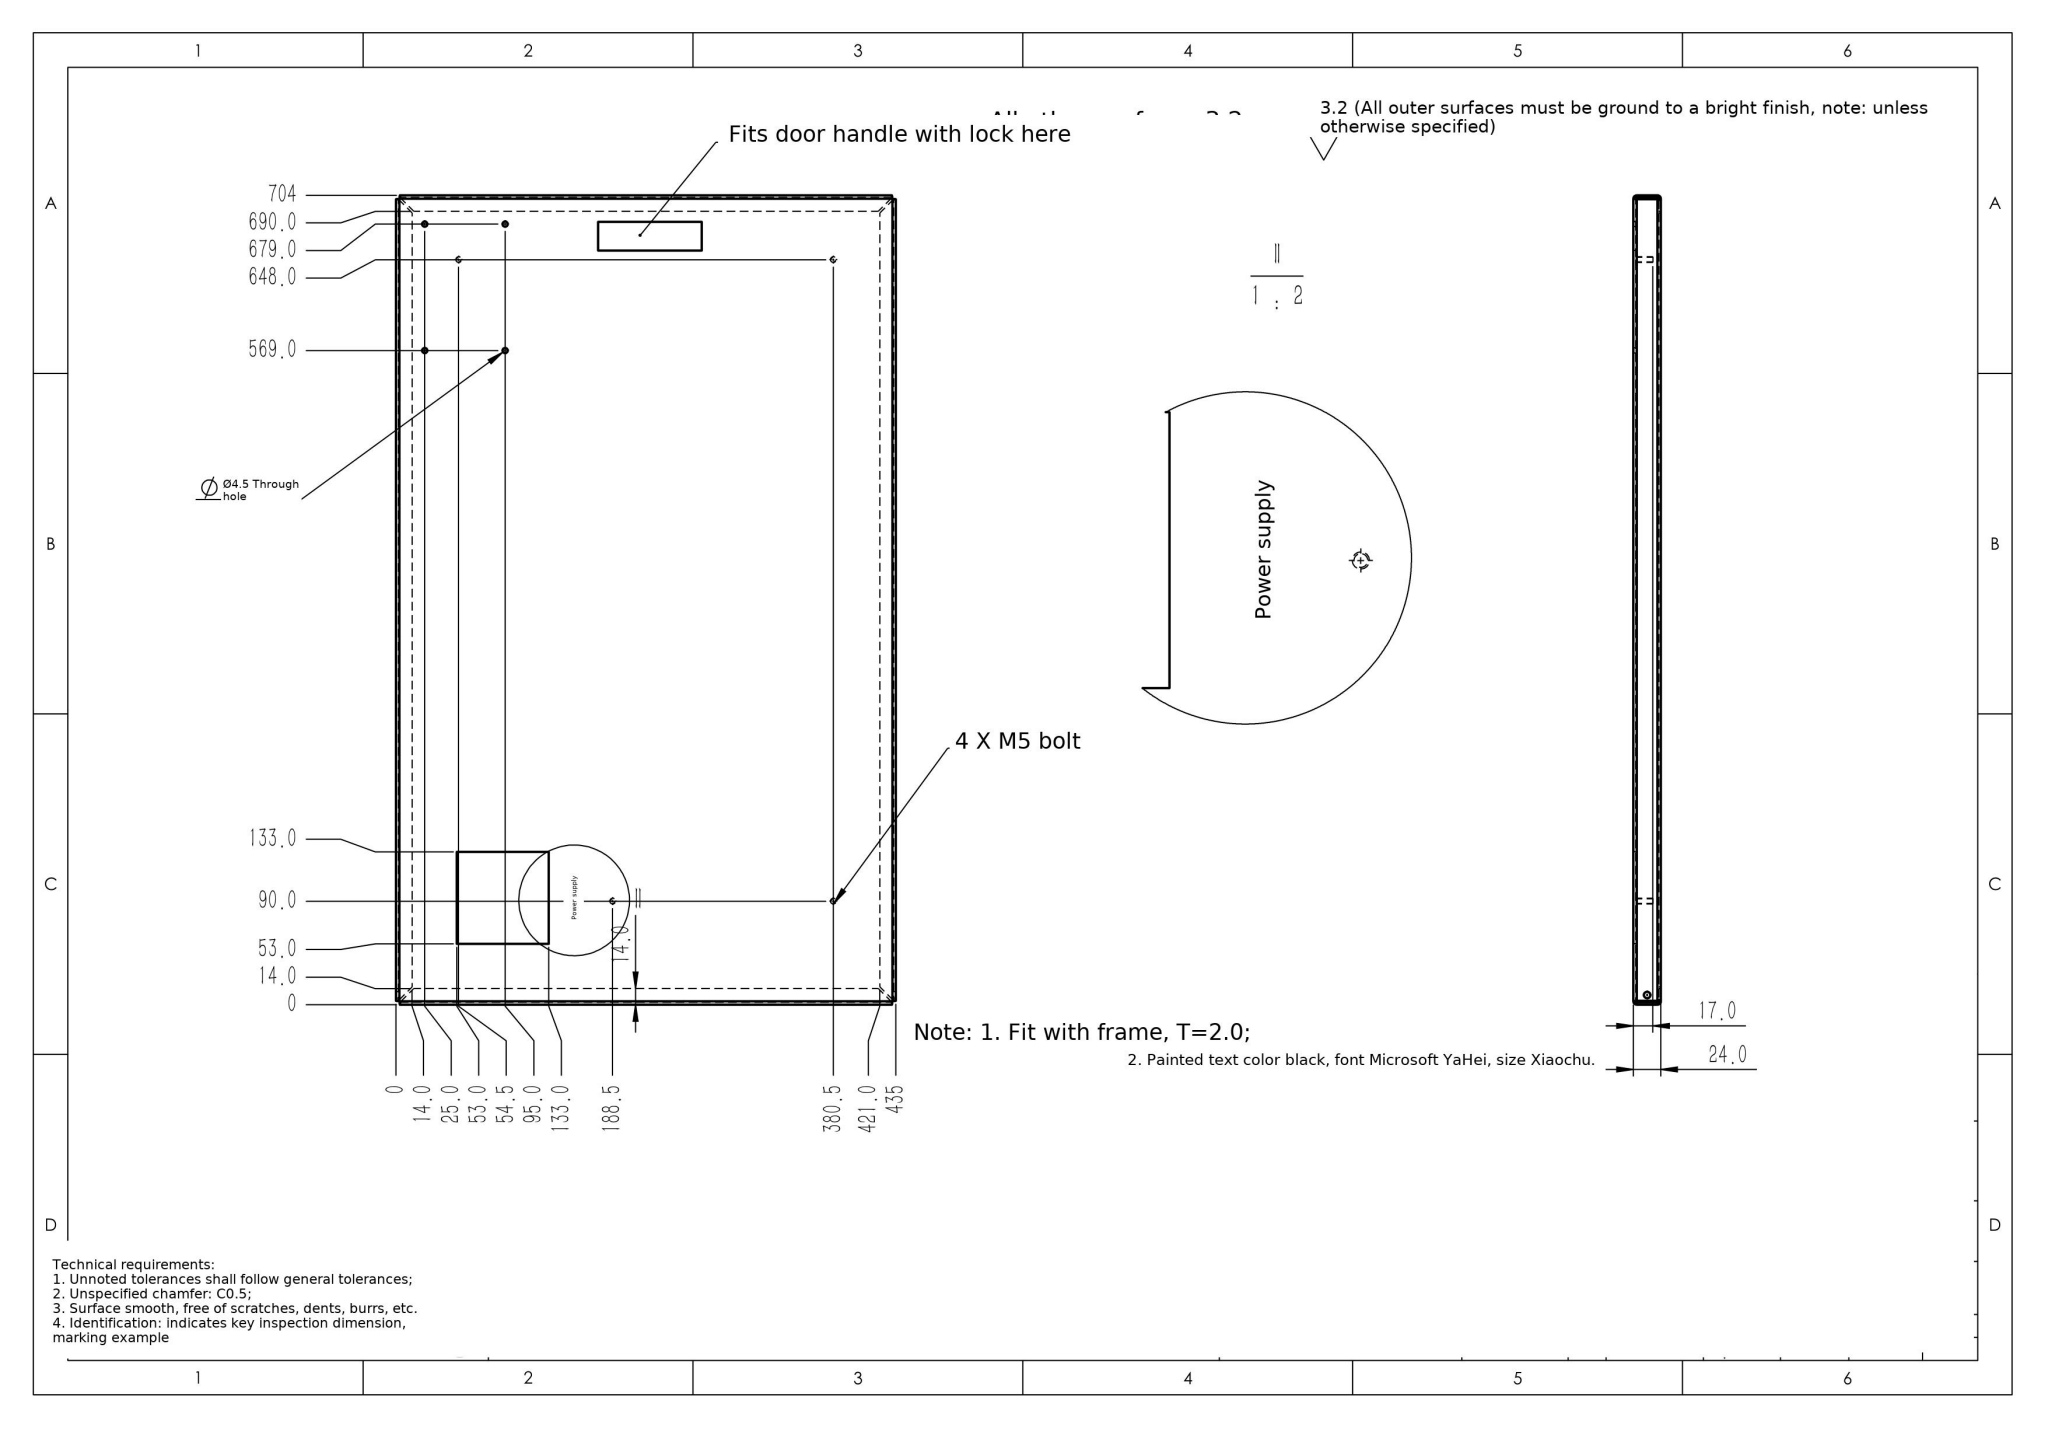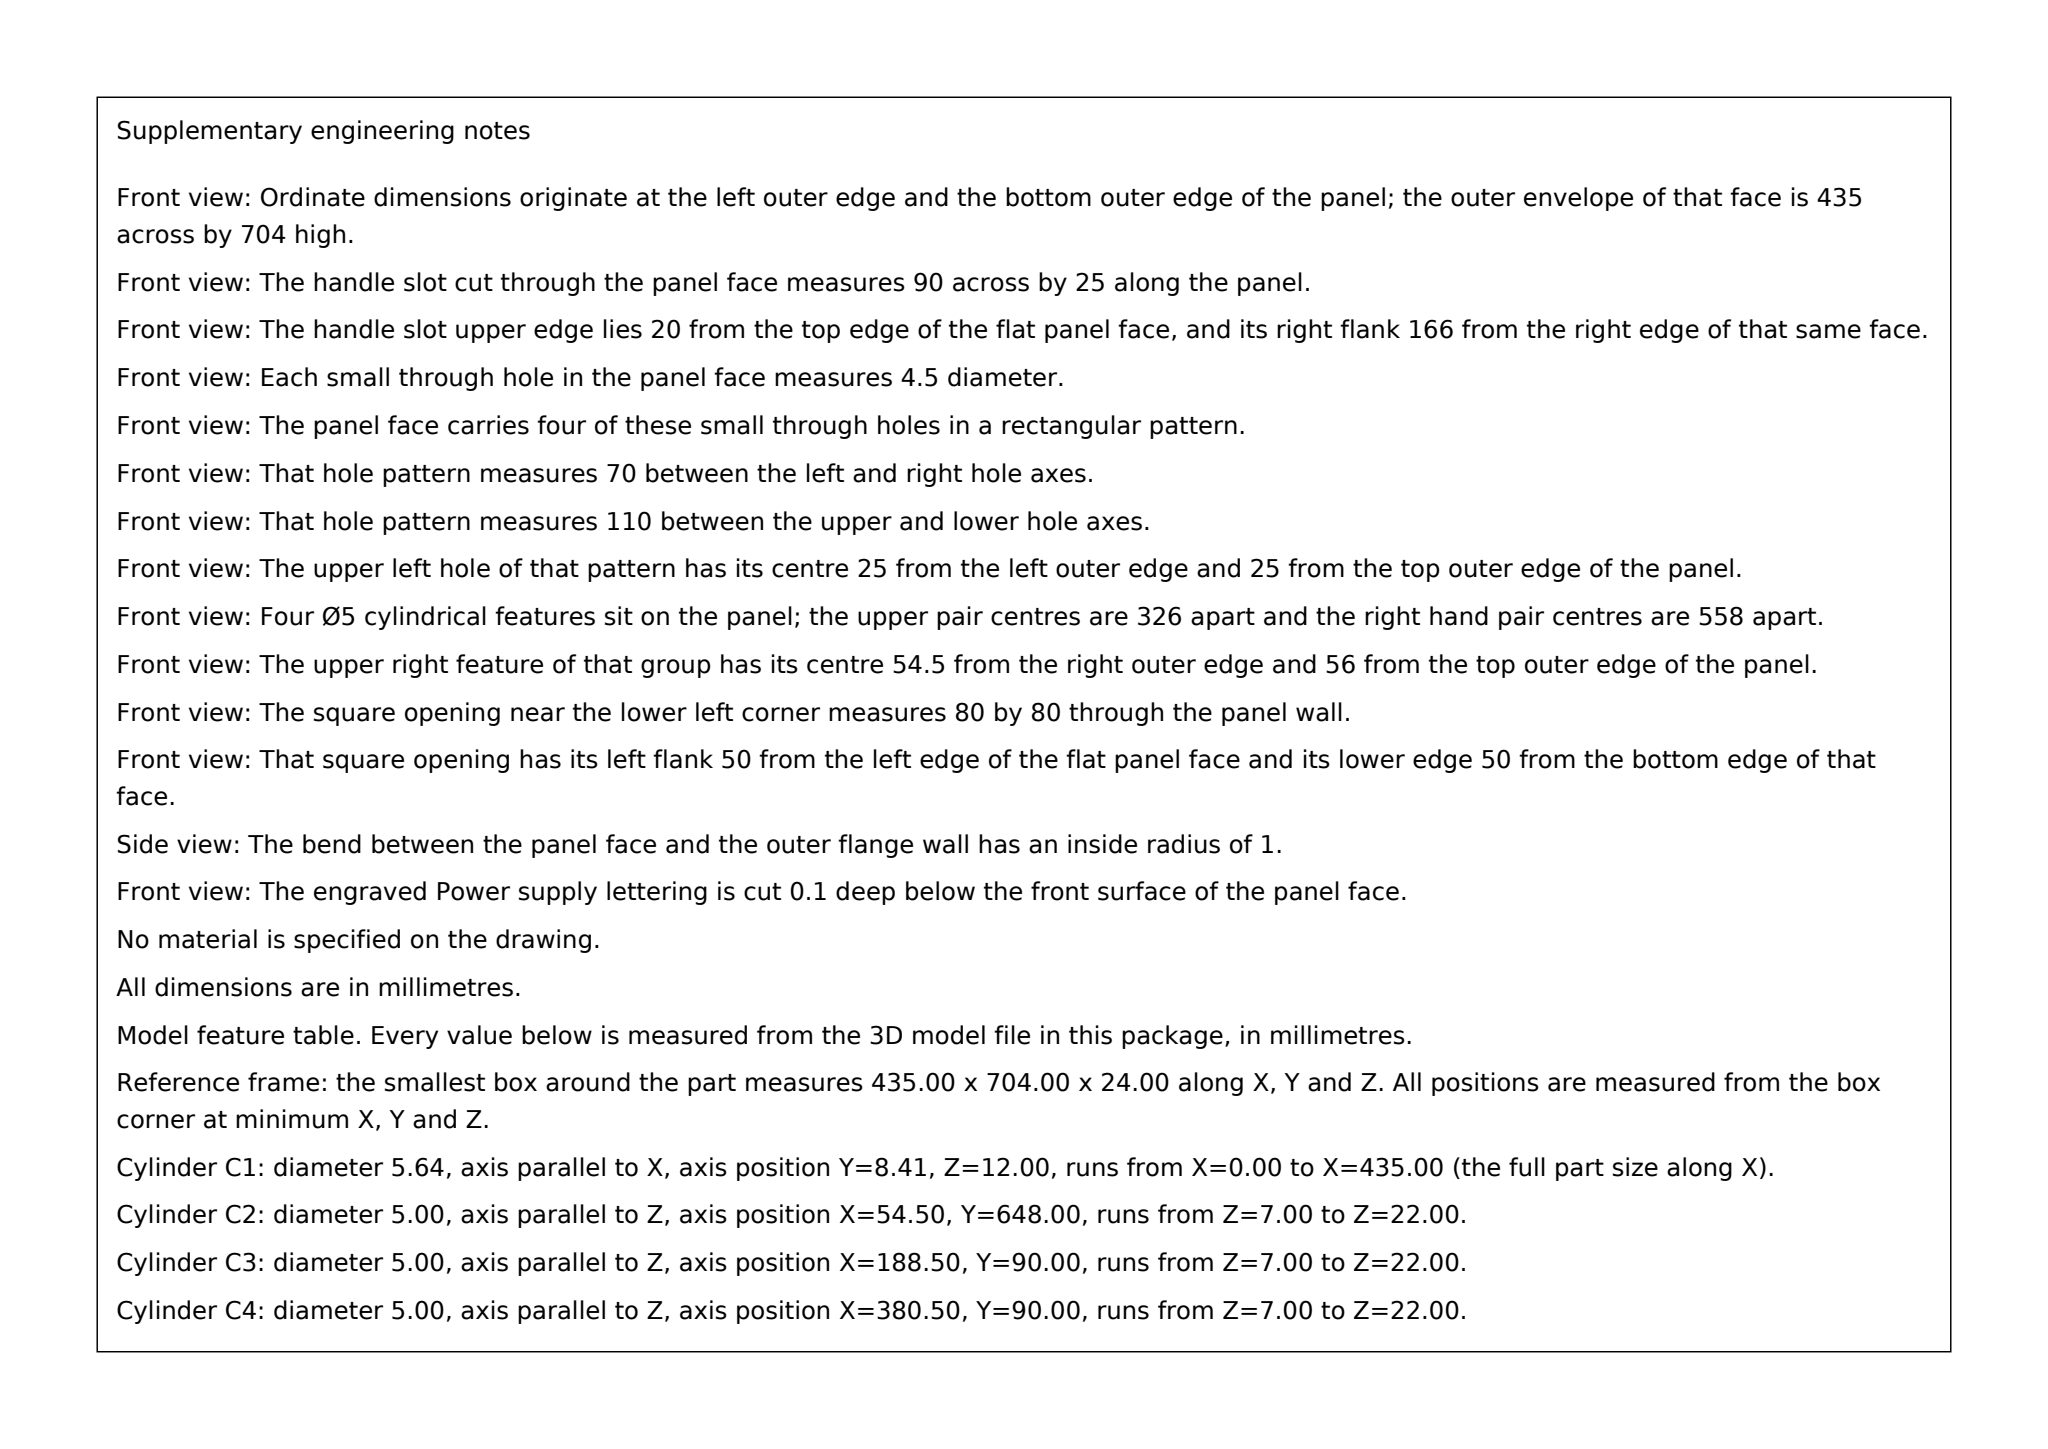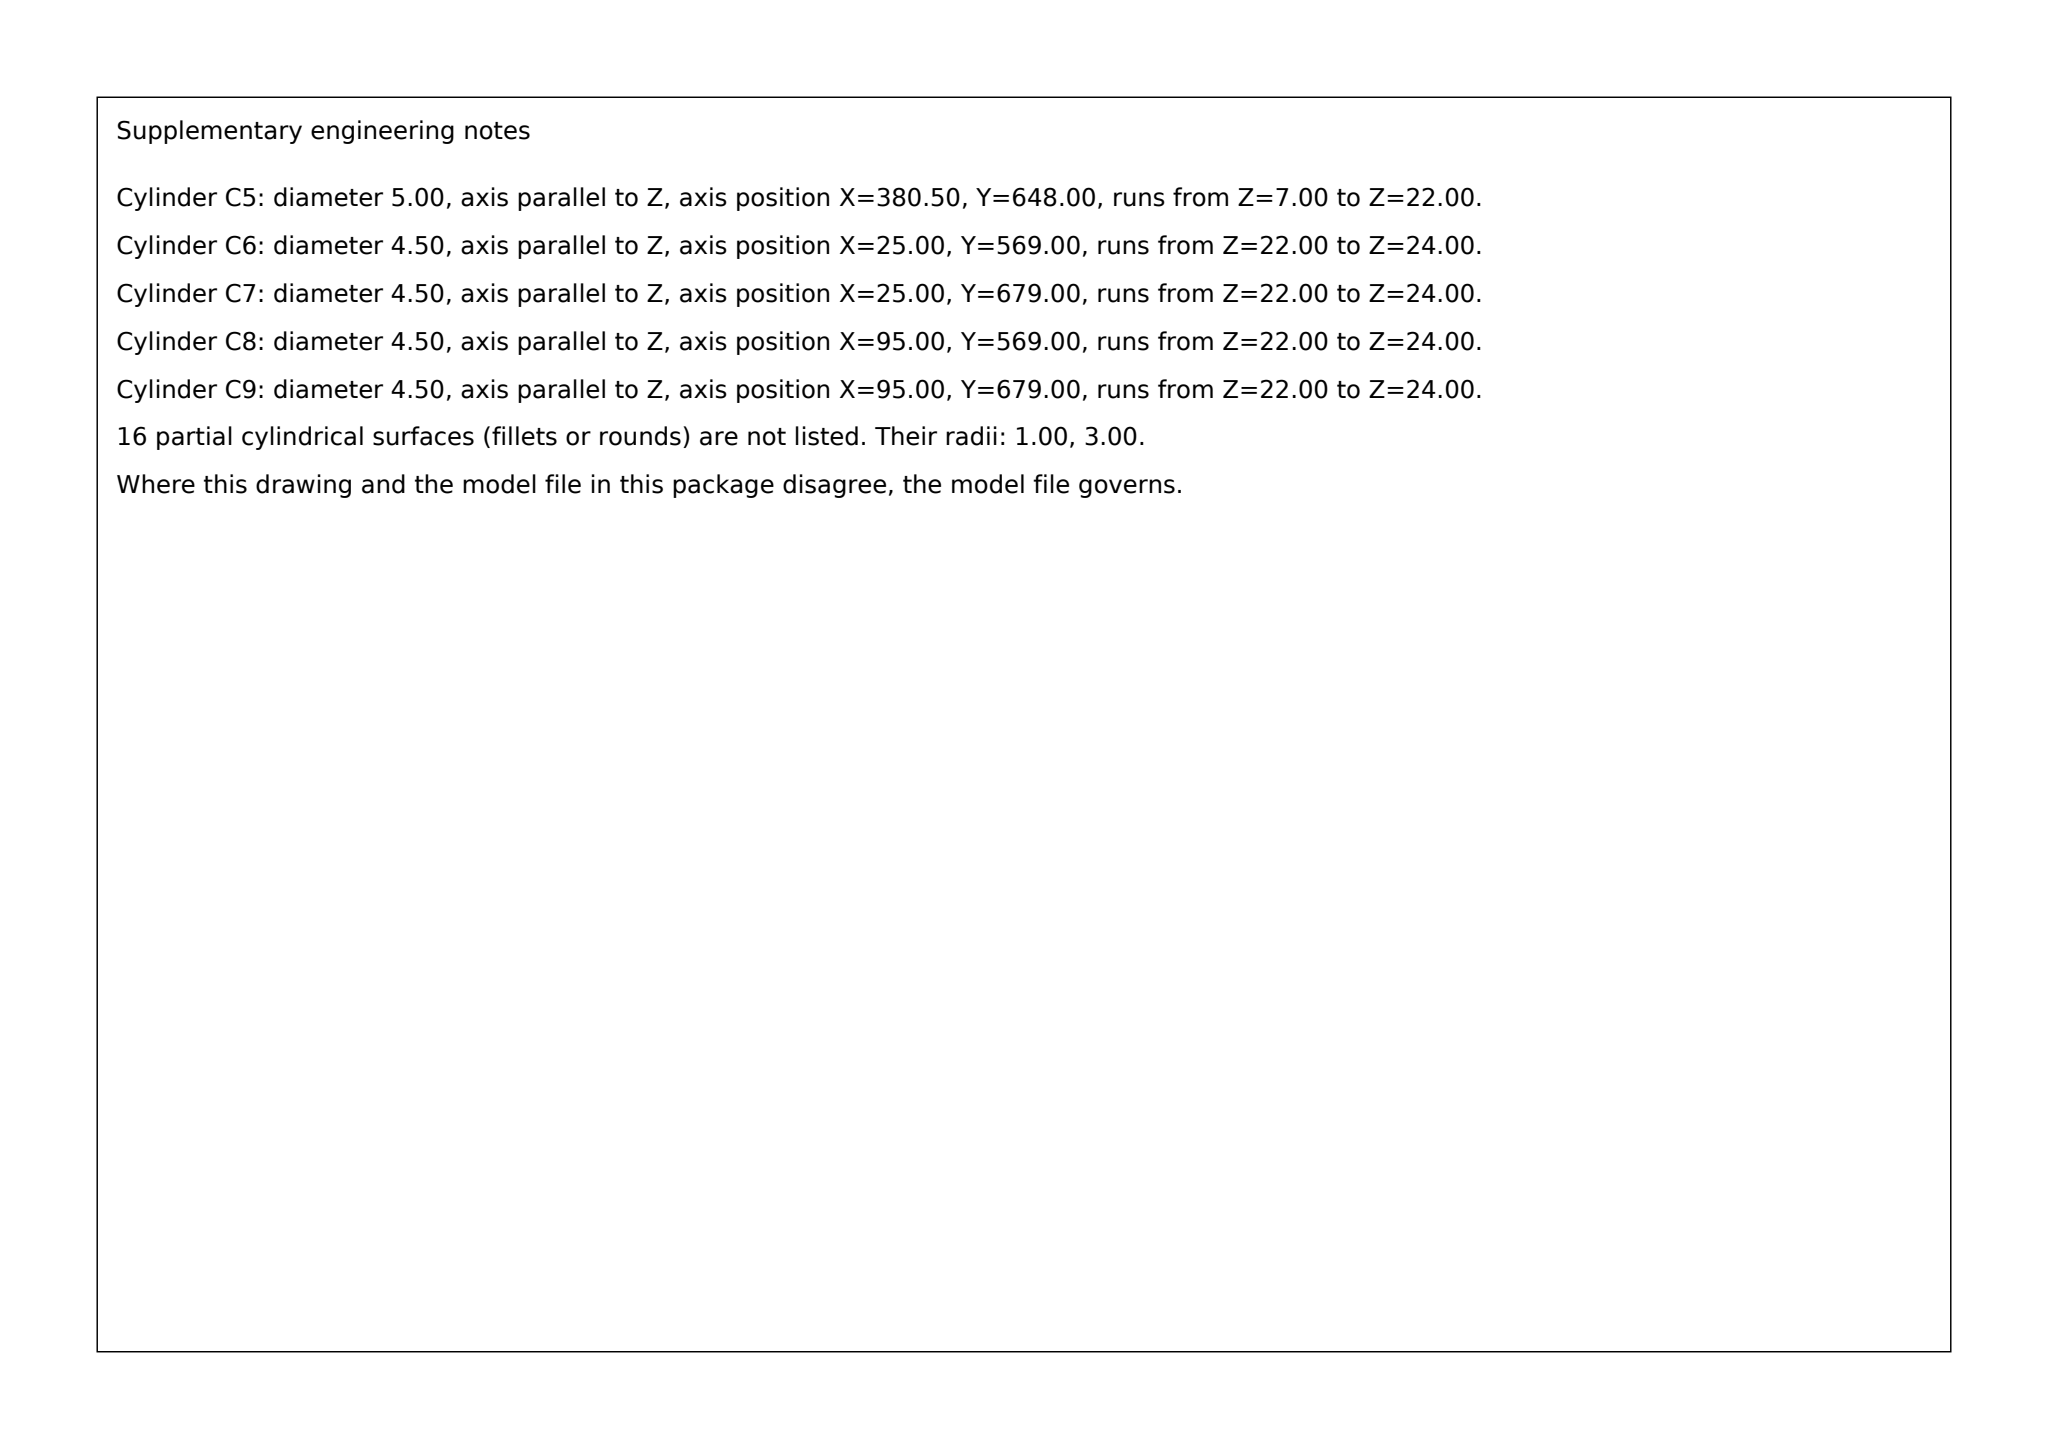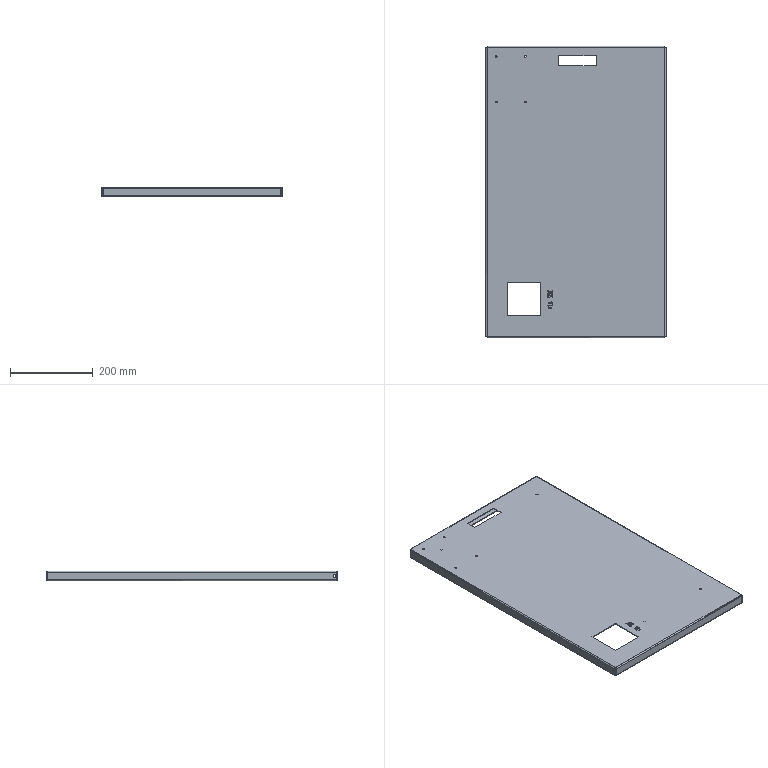Part | SolidWorks | mm | 1 solid | 209 faces | box 435 x 704 x 24 mm | volume 740184 mm3 | plane 128 | spline 45 | cylinder 36 | commonest cylinder face diameters 4.5 x8 5 x8 6 x8 2 x8 5.632 x4
Drawing notes:
POWER SUPPLY PKT 80.0 X 80.0, 53.0 FROM LH & BOTTOM EDGES | from the solid: x planes 53.02 & 133.02, y planes 53.02 & 133.02 = 80 x 80 pocket, 53 from datum edges
4X M5 STUD: 15 LG, PROJ 15 FROM PANEL FACE | from the solid: Ø5.0 z-axis cylinders, length 15.0, from z=7.02 to z=22.02 (panel face z=7.02)
'POWER SUPPLY' AREA 80.0 X 80.0 ENGRAVED DP 0.1 | from the solid: x planes 53.02/133.02 and y planes 53.02/133.02 (80 sq); z planes 23.92 vs 24.02 = 0.1 deep
ENGRAVED "POWER SUPPLY": 41.6 LG X 12.6 HI, ROT 90 (READS UP) | from the solid: x planes 148.64-161.22 (12.58 hi), y planes 72.03-113.65 (41.62 lg)
TEXT ENVELOPE 148.6 FROM LH EDGE, 72.0 FROM BOTTOM EDGE | from the solid: text min corner at x=148.64, y=72.03 from bbox min (LH/bottom edges)
ENGRAVE TEXT 0.1 DP FROM OUTER FACE | from the solid: z planes 23.92 vs face 24.02